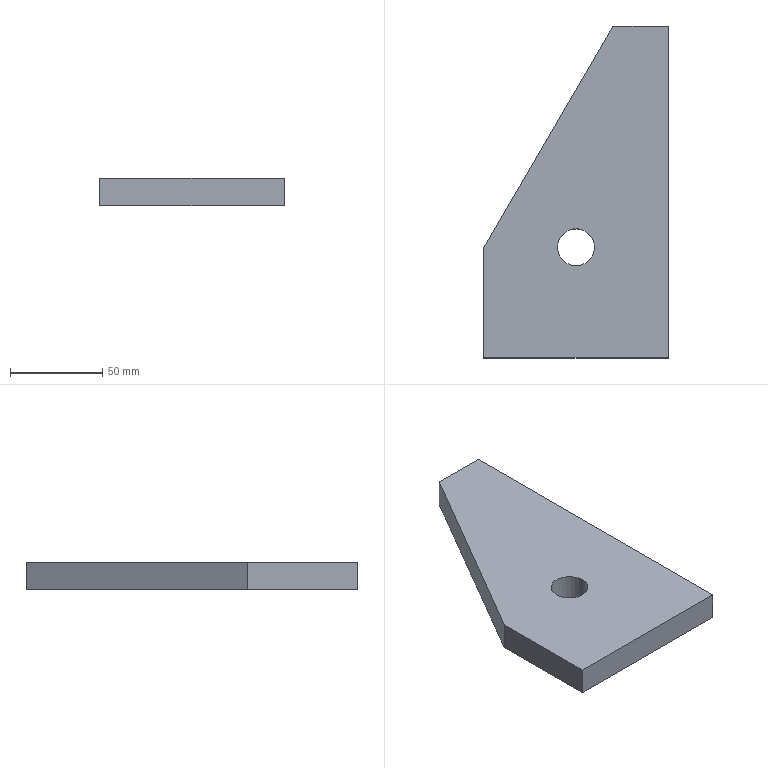Component | SolidWorks | JF21-80.1-1-3(_)-1-SOLID42-1 | 1 solid | 9 faces | box 100 x 180 x 15 mm | volume 202288 mm3 | plane 7 | cylinder 2 | commonest cylinder face diameters 20 x2
STEP:
#1=CARTESIAN_POINT('',(-18.898,-86.22,49.803));
#2=VERTEX_POINT('',#1);
#3=CARTESIAN_POINT('',(-19.685,-86.22,49.803));
#4=VERTEX_POINT('',#3);
#5=CARTESIAN_POINT('',(-19.291,-86.22,49.803));
#6=DIRECTION('',(0.,0.,-1.));
#7=DIRECTION('',(1.,0.,0.));
#8=AXIS2_PLACEMENT_3D('',#5,#6,#7);
#9=CIRCLE('',#8,0.3937);
#10=EDGE_CURVE('',#2,#4,#9,.T.);
#11=ORIENTED_EDGE('',*,*,#10,.T.);
#12=CARTESIAN_POINT('',(-19.685,-86.22,50.394));
#13=VERTEX_POINT('',#12);
#14=CARTESIAN_POINT('',(-19.685,-86.22,-9.843));
#15=DIRECTION('',(0.,0.,1.));
#16=VECTOR('',#15,39.37);
#17=LINE('',#14,#16);
#18=EDGE_CURVE('',#4,#13,#17,.T.);
#19=ORIENTED_EDGE('',*,*,#18,.T.);
#20=CARTESIAN_POINT('',(-18.898,-86.22,50.394));
#21=VERTEX_POINT('',#20);
#22=CARTESIAN_POINT('',(-19.291,-86.22,50.394));
#23=DIRECTION('',(0.,0.,1.));
#24=DIRECTION('',(1.,0.,0.));
#25=AXIS2_PLACEMENT_3D('',#22,#23,#24);
#26=CIRCLE('',#25,0.3937);
#27=EDGE_CURVE('',#13,#21,#26,.T.);
#28=ORIENTED_EDGE('',*,*,#27,.T.);
#29=CARTESIAN_POINT('',(-18.898,-86.22,-9.843));
#30=DIRECTION('',(0.,0.,1.));
#31=VECTOR('',#30,39.37);
#32=LINE('',#29,#31);
#33=EDGE_CURVE('',#2,#21,#32,.T.);
#34=ORIENTED_EDGE('',*,*,#33,.F.);
#35=EDGE_LOOP('',(#11,#19,#28,#34));
#36=FACE_OUTER_BOUND('',#35,.T.);
#37=CARTESIAN_POINT('',(-19.291,-86.22,-9.843));
#38=DIRECTION('',(0.,0.,1.));
#39=DIRECTION('',(-1.,0.,0.));
#40=AXIS2_PLACEMENT_3D('',#37,#38,#39);
#41=CYLINDRICAL_SURFACE('',#40,0.3937);
#42=ADVANCED_FACE('',(#36),#41,.F.);
#43=CARTESIAN_POINT('',(-21.26,-88.583,50.394));
#44=VERTEX_POINT('',#43);
#45=CARTESIAN_POINT('',(-17.323,-88.583,50.394));
#46=VERTEX_POINT('',#45);
#47=CARTESIAN_POINT('',(-21.26,-88.583,50.394));
#48=DIRECTION('',(1.,0.,0.));
#49=VECTOR('',#48,39.37);
#50=LINE('',#47,#49);
#51=EDGE_CURVE('',#44,#46,#50,.T.);
#52=ORIENTED_EDGE('',*,*,#51,.F.);
#53=CARTESIAN_POINT('',(-21.26,-88.583,49.803));
#54=VERTEX_POINT('',#53);
#55=CARTESIAN_POINT('',(-21.26,-88.583,49.803));
#56=DIRECTION('',(0.,0.,1.));
#57=VECTOR('',#56,39.37);
#58=LINE('',#55,#57);
#59=EDGE_CURVE('',#54,#44,#58,.T.);
#60=ORIENTED_EDGE('',*,*,#59,.F.);
#61=CARTESIAN_POINT('',(-17.323,-88.583,49.803));
#62=VERTEX_POINT('',#61);
#63=CARTESIAN_POINT('',(-21.26,-88.583,49.803));
#64=DIRECTION('',(1.,0.,0.));
#65=VECTOR('',#64,39.37);
#66=LINE('',#63,#65);
#67=EDGE_CURVE('',#54,#62,#66,.T.);
#68=ORIENTED_EDGE('',*,*,#67,.T.);
#69=CARTESIAN_POINT('',(-17.323,-88.583,49.803));
#70=DIRECTION('',(0.,0.,1.));
#71=VECTOR('',#70,39.37);
#72=LINE('',#69,#71);
#73=EDGE_CURVE('',#62,#46,#72,.T.);
#74=ORIENTED_EDGE('',*,*,#73,.T.);
#75=EDGE_LOOP('',(#52,#60,#68,#74));
#76=FACE_OUTER_BOUND('',#75,.T.);
#77=CARTESIAN_POINT('',(-21.26,-88.583,49.803));
#78=DIRECTION('',(0.,-1.,0.));
#79=DIRECTION('',(0.,0.,1.));
#80=AXIS2_PLACEMENT_3D('',#77,#78,#79);
#81=PLANE('',#80);
#82=ADVANCED_FACE('',(#76),#81,.T.);
#83=CARTESIAN_POINT('',(-21.26,-86.22,50.394));
#84=VERTEX_POINT('',#83);
#85=CARTESIAN_POINT('',(-21.26,-86.22,50.394));
#86=DIRECTION('',(0.,-1.,0.));
#87=VECTOR('',#86,39.37);
#88=LINE('',#85,#87);
#89=EDGE_CURVE('',#84,#44,#88,.T.);
#90=ORIENTED_EDGE('',*,*,#89,.F.);
#91=CARTESIAN_POINT('',(-21.26,-86.22,49.803));
#92=VERTEX_POINT('',#91);
#93=CARTESIAN_POINT('',(-21.26,-86.22,49.803));
#94=DIRECTION('',(0.,0.,1.));
#95=VECTOR('',#94,39.37);
#96=LINE('',#93,#95);
#97=EDGE_CURVE('',#92,#84,#96,.T.);
#98=ORIENTED_EDGE('',*,*,#97,.F.);
#99=CARTESIAN_POINT('',(-21.26,-86.22,49.803));
#100=DIRECTION('',(0.,-1.,0.));
#101=VECTOR('',#100,39.37);
#102=LINE('',#99,#101);
#103=EDGE_CURVE('',#92,#54,#102,.T.);
#104=ORIENTED_EDGE('',*,*,#103,.T.);
#105=ORIENTED_EDGE('',*,*,#59,.T.);
#106=EDGE_LOOP('',(#90,#98,#104,#105));
#107=FACE_OUTER_BOUND('',#106,.T.);
#108=CARTESIAN_POINT('',(-21.26,-86.22,49.803));
#109=DIRECTION('',(-1.,0.,0.));
#110=DIRECTION('',(0.,0.,-1.));
#111=AXIS2_PLACEMENT_3D('',#108,#109,#110);
#112=PLANE('',#111);
#113=ADVANCED_FACE('',(#107),#112,.T.);
#114=CARTESIAN_POINT('',(-18.504,-81.496,50.394));
#115=VERTEX_POINT('',#114);
#116=CARTESIAN_POINT('',(-18.504,-81.496,50.394));
#117=DIRECTION('',(-0.5039,-0.8638,0.));
#118=VECTOR('',#117,39.37);
#119=LINE('',#116,#118);
#120=EDGE_CURVE('',#115,#84,#119,.T.);
#121=ORIENTED_EDGE('',*,*,#120,.F.);
#122=CARTESIAN_POINT('',(-18.504,-81.496,49.803));
#123=VERTEX_POINT('',#122);
#124=CARTESIAN_POINT('',(-18.504,-81.496,49.803));
#125=DIRECTION('',(0.,0.,1.));
#126=VECTOR('',#125,39.37);
#127=LINE('',#124,#126);
#128=EDGE_CURVE('',#123,#115,#127,.T.);
#129=ORIENTED_EDGE('',*,*,#128,.F.);
#130=CARTESIAN_POINT('',(-18.504,-81.496,49.803));
#131=DIRECTION('',(-0.5039,-0.8638,0.));
#132=VECTOR('',#131,39.37);
#133=LINE('',#130,#132);
#134=EDGE_CURVE('',#123,#92,#133,.T.);
#135=ORIENTED_EDGE('',*,*,#134,.T.);
#136=ORIENTED_EDGE('',*,*,#97,.T.);
#137=EDGE_LOOP('',(#121,#129,#135,#136));
#138=FACE_OUTER_BOUND('',#137,.T.);
#139=CARTESIAN_POINT('',(-18.504,-81.496,49.803));
#140=DIRECTION('',(-0.8638,0.5039,0.));
#141=DIRECTION('',(0.5039,0.8638,0.));
#142=AXIS2_PLACEMENT_3D('',#139,#140,#141);
#143=PLANE('',#142);
#144=ADVANCED_FACE('',(#138),#143,.T.);
#145=CARTESIAN_POINT('',(-17.323,-81.496,50.394));
#146=VERTEX_POINT('',#145);
#147=CARTESIAN_POINT('',(-17.323,-81.496,50.394));
#148=DIRECTION('',(-1.,0.,0.));
#149=VECTOR('',#148,39.37);
#150=LINE('',#147,#149);
#151=EDGE_CURVE('',#146,#115,#150,.T.);
#152=ORIENTED_EDGE('',*,*,#151,.F.);
#153=CARTESIAN_POINT('',(-17.323,-81.496,49.803));
#154=VERTEX_POINT('',#153);
#155=CARTESIAN_POINT('',(-17.323,-81.496,49.803));
#156=DIRECTION('',(0.,0.,1.));
#157=VECTOR('',#156,39.37);
#158=LINE('',#155,#157);
#159=EDGE_CURVE('',#154,#146,#158,.T.);
#160=ORIENTED_EDGE('',*,*,#159,.F.);
#161=CARTESIAN_POINT('',(-17.323,-81.496,49.803));
#162=DIRECTION('',(-1.,0.,0.));
#163=VECTOR('',#162,39.37);
#164=LINE('',#161,#163);
#165=EDGE_CURVE('',#154,#123,#164,.T.);
#166=ORIENTED_EDGE('',*,*,#165,.T.);
#167=ORIENTED_EDGE('',*,*,#128,.T.);
#168=EDGE_LOOP('',(#152,#160,#166,#167));
#169=FACE_OUTER_BOUND('',#168,.T.);
#170=CARTESIAN_POINT('',(-17.323,-81.496,49.803));
#171=DIRECTION('',(0.,1.,0.));
#172=DIRECTION('',(0.,0.,-1.));
#173=AXIS2_PLACEMENT_3D('',#170,#171,#172);
#174=PLANE('',#173);
#175=ADVANCED_FACE('',(#169),#174,.T.);
#176=CARTESIAN_POINT('',(-17.323,-88.583,50.394));
#177=DIRECTION('',(0.,1.,0.));
#178=VECTOR('',#177,39.37);
#179=LINE('',#176,#178);
#180=EDGE_CURVE('',#46,#146,#179,.T.);
#181=ORIENTED_EDGE('',*,*,#180,.F.);
#182=ORIENTED_EDGE('',*,*,#73,.F.);
#183=CARTESIAN_POINT('',(-17.323,-88.583,49.803));
#184=DIRECTION('',(0.,1.,0.));
#185=VECTOR('',#184,39.37);
#186=LINE('',#183,#185);
#187=EDGE_CURVE('',#62,#154,#186,.T.);
#188=ORIENTED_EDGE('',*,*,#187,.T.);
#189=ORIENTED_EDGE('',*,*,#159,.T.);
#190=EDGE_LOOP('',(#181,#182,#188,#189));
#191=FACE_OUTER_BOUND('',#190,.T.);
#192=CARTESIAN_POINT('',(-17.323,-88.583,49.803));
#193=DIRECTION('',(1.,0.,0.));
#194=DIRECTION('',(0.,0.,1.));
#195=AXIS2_PLACEMENT_3D('',#192,#193,#194);
#196=PLANE('',#195);
#197=ADVANCED_FACE('',(#191),#196,.T.);
#198=ORIENTED_EDGE('',*,*,#10,.F.);
#199=CARTESIAN_POINT('',(-19.291,-86.22,49.803));
#200=DIRECTION('',(0.,0.,-1.));
#201=DIRECTION('',(1.,0.,0.));
#202=AXIS2_PLACEMENT_3D('',#199,#200,#201);
#203=CIRCLE('',#202,0.3937);
#204=EDGE_CURVE('',#4,#2,#203,.T.);
#205=ORIENTED_EDGE('',*,*,#204,.F.);
#206=EDGE_LOOP('',(#198,#205));
#207=FACE_BOUND('',#206,.T.);
#208=ORIENTED_EDGE('',*,*,#67,.F.);
#209=ORIENTED_EDGE('',*,*,#103,.F.);
#210=ORIENTED_EDGE('',*,*,#134,.F.);
#211=ORIENTED_EDGE('',*,*,#165,.F.);
#212=ORIENTED_EDGE('',*,*,#187,.F.);
#213=EDGE_LOOP('',(#208,#209,#210,#211,#212));
#214=FACE_OUTER_BOUND('',#213,.T.);
#215=CARTESIAN_POINT('',(-17.323,-88.583,49.803));
#216=DIRECTION('',(0.,0.,1.));
#217=DIRECTION('',(-1.,0.,0.));
#218=AXIS2_PLACEMENT_3D('',#215,#216,#217);
#219=PLANE('',#218);
#220=ADVANCED_FACE('',(#207,#214),#219,.F.);
#221=CARTESIAN_POINT('',(-19.291,-86.22,50.394));
#222=DIRECTION('',(0.,0.,1.));
#223=DIRECTION('',(1.,0.,0.));
#224=AXIS2_PLACEMENT_3D('',#221,#222,#223);
#225=CIRCLE('',#224,0.3937);
#226=EDGE_CURVE('',#21,#13,#225,.T.);
#227=ORIENTED_EDGE('',*,*,#226,.F.);
#228=ORIENTED_EDGE('',*,*,#27,.F.);
#229=EDGE_LOOP('',(#227,#228));
#230=FACE_BOUND('',#229,.T.);
#231=ORIENTED_EDGE('',*,*,#51,.T.);
#232=ORIENTED_EDGE('',*,*,#180,.T.);
#233=ORIENTED_EDGE('',*,*,#151,.T.);
#234=ORIENTED_EDGE('',*,*,#120,.T.);
#235=ORIENTED_EDGE('',*,*,#89,.T.);
#236=EDGE_LOOP('',(#231,#232,#233,#234,#235));
#237=FACE_OUTER_BOUND('',#236,.T.);
#238=CARTESIAN_POINT('',(-17.323,-88.583,50.394));
#239=DIRECTION('',(0.,0.,1.));
#240=DIRECTION('',(-1.,0.,0.));
#241=AXIS2_PLACEMENT_3D('',#238,#239,#240);
#242=PLANE('',#241);
#243=ADVANCED_FACE('',(#230,#237),#242,.T.);
#244=ORIENTED_EDGE('',*,*,#18,.F.);
#245=ORIENTED_EDGE('',*,*,#204,.T.);
#246=ORIENTED_EDGE('',*,*,#33,.T.);
#247=ORIENTED_EDGE('',*,*,#226,.T.);
#248=EDGE_LOOP('',(#244,#245,#246,#247));
#249=FACE_OUTER_BOUND('',#248,.T.);
#250=CARTESIAN_POINT('',(-19.291,-86.22,-9.843));
#251=DIRECTION('',(0.,0.,1.));
#252=DIRECTION('',(-1.,0.,0.));
#253=AXIS2_PLACEMENT_3D('',#250,#251,#252);
#254=CYLINDRICAL_SURFACE('',#253,0.3937);
#255=ADVANCED_FACE('',(#249),#254,.F.);
#256=CLOSED_SHELL('',(#42,#82,#113,#144,#175,#197,#220,#243,#255));
#257=MANIFOLD_SOLID_BREP('',#256);
#258=CARTESIAN_POINT('',(0.,0.,0.));
#259=DIRECTION('',(0.,0.,1.));
#260=DIRECTION('',(1.,0.,0.));
#261=AXIS2_PLACEMENT_3D('',#258,#259,#260);
#262=(LENGTH_UNIT()NAMED_UNIT(*)SI_UNIT($,.METRE.));
#263=LENGTH_MEASURE_WITH_UNIT(LENGTH_MEASURE(0.0254),#262);
#264=DIMENSIONAL_EXPONENTS(1.,0.,0.,0.,0.,0.,0.);
#265=(CONVERSION_BASED_UNIT('',#263)LENGTH_UNIT()NAMED_UNIT(#264));
#266=UNCERTAINTY_MEASURE_WITH_UNIT(LENGTH_MEASURE(0.00001),#265,'','');
#267=(NAMED_UNIT(*)PLANE_ANGLE_UNIT()SI_UNIT($,.RADIAN.));
#268=(NAMED_UNIT(*)SI_UNIT($,.STERADIAN.)SOLID_ANGLE_UNIT());
#269=(GEOMETRIC_REPRESENTATION_CONTEXT(3)GLOBAL_UNCERTAINTY_ASSIGNED_CONTEXT((#266))GLOBAL_UNIT_ASSIGNED_CONTEXT((#265,#267,#268))REPRESENTATION_CONTEXT('',''));
#270=ADVANCED_BREP_SHAPE_REPRESENTATION('',(#257,#261),#269);
#271=COLOUR_RGB('',0.7922,0.8196,0.9333);
#272=FILL_AREA_STYLE_COLOUR('',#271);
#273=FILL_AREA_STYLE('',(#272));
#274=SURFACE_STYLE_FILL_AREA(#273);
#275=SURFACE_SIDE_STYLE('',(#274));
#276=SURFACE_STYLE_USAGE(.BOTH.,#275);
#277=PRESENTATION_STYLE_ASSIGNMENT((#276));
#278=STYLED_ITEM('',(#277),#257);
#279=(LENGTH_UNIT()NAMED_UNIT(*)SI_UNIT($,.METRE.));
#280=LENGTH_MEASURE_WITH_UNIT(LENGTH_MEASURE(0.0254),#279);
#281=DIMENSIONAL_EXPONENTS(1.,0.,0.,0.,0.,0.,0.);
#282=(CONVERSION_BASED_UNIT('',#280)LENGTH_UNIT()NAMED_UNIT(#281));
#283=UNCERTAINTY_MEASURE_WITH_UNIT(LENGTH_MEASURE(0.00001),#282,'','');
#284=(NAMED_UNIT(*)PLANE_ANGLE_UNIT()SI_UNIT($,.RADIAN.));
#285=(NAMED_UNIT(*)SI_UNIT($,.STERADIAN.)SOLID_ANGLE_UNIT());
#286=(GEOMETRIC_REPRESENTATION_CONTEXT(3)GLOBAL_UNCERTAINTY_ASSIGNED_CONTEXT((#283))GLOBAL_UNIT_ASSIGNED_CONTEXT((#282,#284,#285))REPRESENTATION_CONTEXT('',''));
#287=MECHANICAL_DESIGN_GEOMETRIC_PRESENTATION_REPRESENTATION('',(#278),#286);
#288=PRESENTATION_LAYER_ASSIGNMENT('','',(#278));